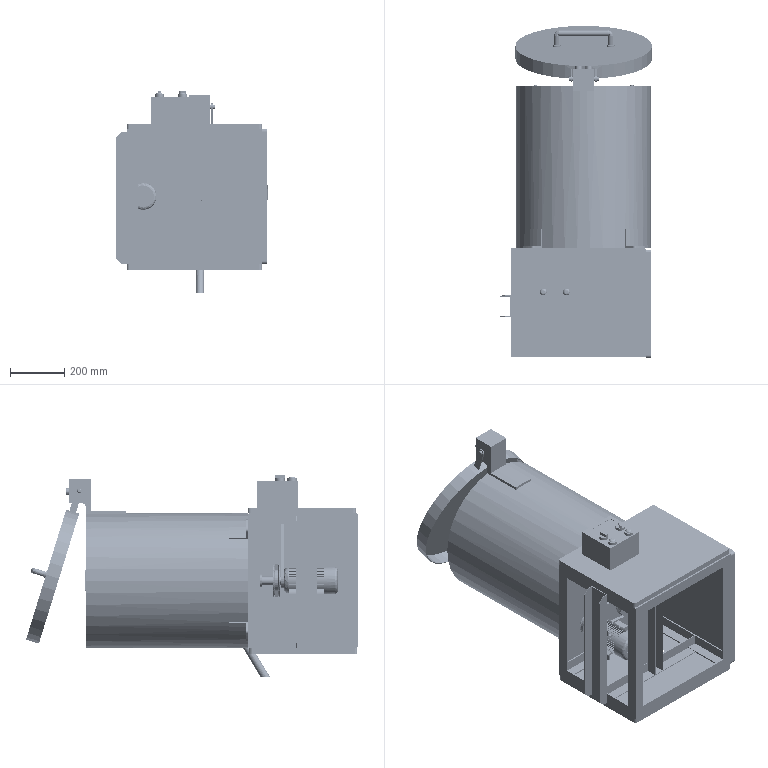Assembly | SolidWorks | mm | 25 component files | 25 solids | 4277 faces | box 563 x 1229.75 x 749.72 mm | volume 23882375 mm3 | cylinder 3555 | plane 692 | cone 12 | spline 10 | torus 8 | commonest cylinder face diameters 3 x3240 20 x39 30 x17 13.811 x16 6 x16 42.675 x13 366.053 x13 10 x12
Bill of materials:
FilterScreen | 1 |  | Closed cylindrical drum with a perforated curved wall, a central hole in one flat end, and a small U-shaped loop or bracket on the other end.
Housing | 1 |  | Cylindrical housing with six radial tabs around one end, a raised round boss with a small central hole on that end face, a block bracket with a hole and a pin on top, and a slanted rod sticking out below.
Lid | 1 |  | Shallow round disc or lid with a raised rim, a U-shaped tubular handle on one face, and two flat tabs with holes sticking out from the edge.
LX-TSJ-02 | 2 |  | Square flange with rounded corners and four corner holes, with a two-step cylindrical boss and a central through-bore.
LX-TSJ-03 | 1 |  | Open box-shaped frame made of square-section bars along all twelve edges, with one side closed by a panel that has a large round hole.
LX-TSJ-04 | 1 |  | Grooved wheel (sheave-like) with a trapezoidal groove around its rim, a recessed face, a central bore with one keyway, and five holes around the bore.
LX-TSJ-05 | 1 |  | Cylindrical body with long straight fins in the middle, rounded end caps, a box on one side, and a bent mounting bracket with four holes. Six holes are on one end face. The overall form looks like a motor.
LX-TSJ-07 | 1 |  | Long solid round rod with a thin raised collar near one end and a flat or slot-like cut at that end.
LX-TSJ-08 | 1 |  | Grooved wheel (sheave-like) with a deep trapezoidal groove around its rim, a recessed hub face, a central bore with two keyway notches, and five holes around the bore.
LX-TSJ-09 | 1 |  | Long L-section angle where one leg is cut shorter than the other at both ends.
LX-TSJ-13 | 2 |  | Thin flat closed loop shaped like a tapered oval, with a larger rounded end and a smaller rounded end joined by straight sides.
LX-TSJ-14 | 2 |  | Short L-section angle, shown upright, where one leg is cut shorter than the other at both ends.
LX-TSJ-15 | 2 |  | Long, slender straight prismatic bar with thin walls; one orthographic view shows an L-shaped outline, suggesting an angle (L) cross-section, and another view shows angled cuts at both ends on one side.
LX-TSJ-16 | 1 |  | Thin flat rectangular plate with rounded corners and one rounded-rectangle (obround) through-cutout set toward one corner.
LX-TSJ-16 | 1 |  | Thin, shallow rectangular tray: a flat plate with rounded outer corners and a low wall running around the whole perimeter. One long edge has a small rectangular notch cut through both the wall and the plate. There is also a rounded-rectangle through-opening in the plate, off-center toward the notched edge.
LX-TSJ-17 | 1 |  | Flat rectangular plate with rounded corners and one semicircular notch cut into one long edge.
Part1^CentrifugalDehydrator | 1 |  | Plain solid cylindrical rod with flat square-cut ends.
Part2^CentrifugalDehydrator | 1 |  | Rectangular block with features on its top face: two short cylindrical bosses with domed tops, and two raised D-shaped (half-round) bosses that each have a flat upright wall on one side. A thin line or shallow step runs along part of the top face.
Part3^CentrifugalDehydrator | 1 |  | Thin flat obround (stadium-shaped) closed loop or ring with a long slot-shaped central opening.
Part4^CentrifugalDehydrator | 1 |  | Solid cylindrical pin with chamfered edges at both ends.
Tray | 1 |  | Open cylindrical cage frame: circular end rings and a middle ring joined by axial ribs, with one end closed by a disc that has radial slots arranged around a small central hole.
Mates:
1. coincident | LX-TSJ-03-1 face at (-393.022, -784.978, -164.298) dir (-1, 0, 0) | LX-TSJ-16-1 edge at (-393.022, -768.978, -144.298) dir (0, 1, 0)
2. parallel | LX-TSJ-03-1 face at (-393.022, -784.978, -164.298) dir (0, 0, 1) | LX-TSJ-16-1 face at (96.978, -768.978, -144.298) dir (0, 0, 1)
3. coincident | LX-TSJ-03-1 face at (-393.022, -784.978, -164.298) dir (0, 0, 1) | LX-TSJ-16-1 face at (96.978, -768.978, -164.298) dir (0, 0, -1)
4. coincident | LX-TSJ-03-1 face at (-393.022, -378.978, -164.298) dir (0, 1, 0) | LX-TSJ-16-1 face at (96.978, -378.978, -164.298) dir (0, 1, 0)
5. concentric | FilterScreen-1 face at (-123.022, 191.022, -414.298) dir (0, -1, 0) r 187.386 | Housing-2 face at (-123.022, -378.978, -414.298) dir (0, 1, 0) r 250
6. parallel | Part2^CentrifugalDehydrator-1 face at (-304.449, -414.764, -44.298) dir (-1, 0, 0) | Housing-2 face at (-163.022, 71.022, -167.519) dir (-1, 0, 0)
7. coincident | LX-TSJ-03-1 face at (-393.022, -378.978, -164.298) dir (0, 1, 0) | Housing-2 face at (-123.022, -378.978, -414.298) dir (0, -1, 0)
8. concentric | Housing-2 face at (-215.022, 245.823, -81.841) dir (1, 0, 0) r 8 | Part4^CentrifugalDehydrator-2 face at (-68.022, 245.823, -81.841) dir (-1, 0, 0) r 8
9. width | Part4^CentrifugalDehydrator-2 face at (-178.022, 245.823, -81.841) dir (-1, 0, 0) | Part4^CentrifugalDehydrator-2 face at (-68.022, 245.823, -81.841) dir (1, 0, 0) | Housing-2 face at (-163.022, 71.022, -167.519) dir (-1, 0, 0) | Housing-2 face at (-83.022, 71.022, -167.519) dir (1, 0, 0)
10. concentric | Lid-2 face at (-171.682, 245.823, -81.841) dir (1, 0, 0) r 12.5 | Part4^CentrifugalDehydrator-2 face at (-68.022, 245.823, -81.841) dir (-1, 0, 0) r 8
11. width | Lid-2 face at (-74.362, 368.09, -392.024) dir (1, 0, 0) | Lid-2 face at (-171.682, 368.09, -392.024) dir (-1, 0, 0) | Housing-2 face at (-83.022, 71.022, -167.519) dir (1, 0, 0) | Housing-2 face at (-163.022, 71.022, -167.519) dir (-1, 0, 0)
12. concentric | LX-TSJ-04-1 face at (-123.022, -481.3, -414.298) dir (0, 1, 0) r 42.5 | FilterScreen-1 face at (-123.022, 191.022, -414.298) dir (0, -1, 0) r 187.386
13. distance | FilterScreen-1 face at (-123.022, -358.978, -414.298) dir (0, -1, 0) | LX-TSJ-03-1 face at (-393.022, -378.978, -164.298) dir (0, 1, 0)